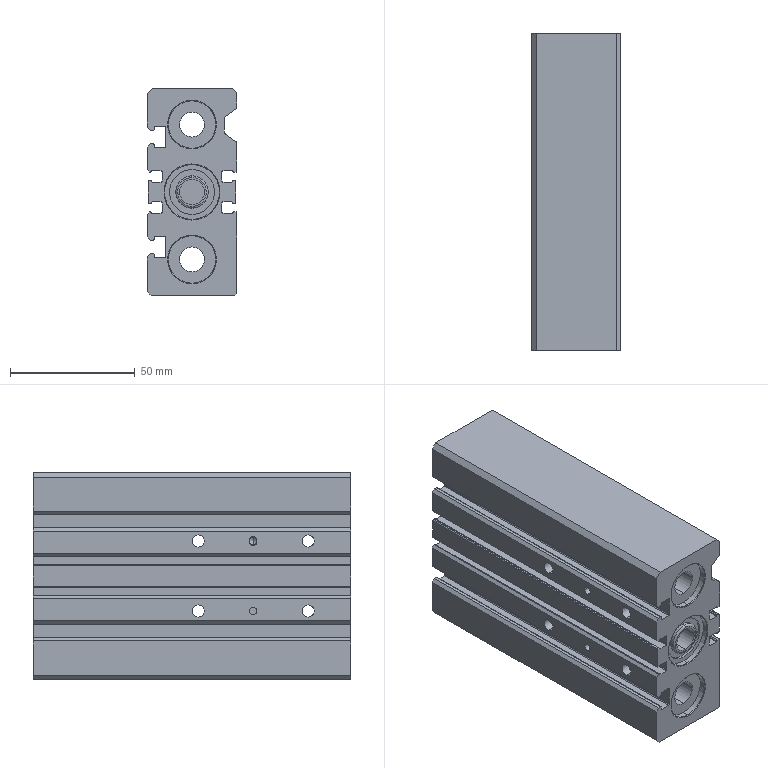Component | SolidWorks | TCL20x90SCylinder-1_TC-L-20x9090_b-1 | 1 solid | 287 faces | volume 266018 mm3 | cylinder 130 | plane 95 | cone 60 | spline 2 | commonest cylinder face diameters 0.8 x20 3 x14 0.4 x12 0.6 x10 4.917 x8 9.5 x8 4.134 x8 5.5 x8 | material SKD11